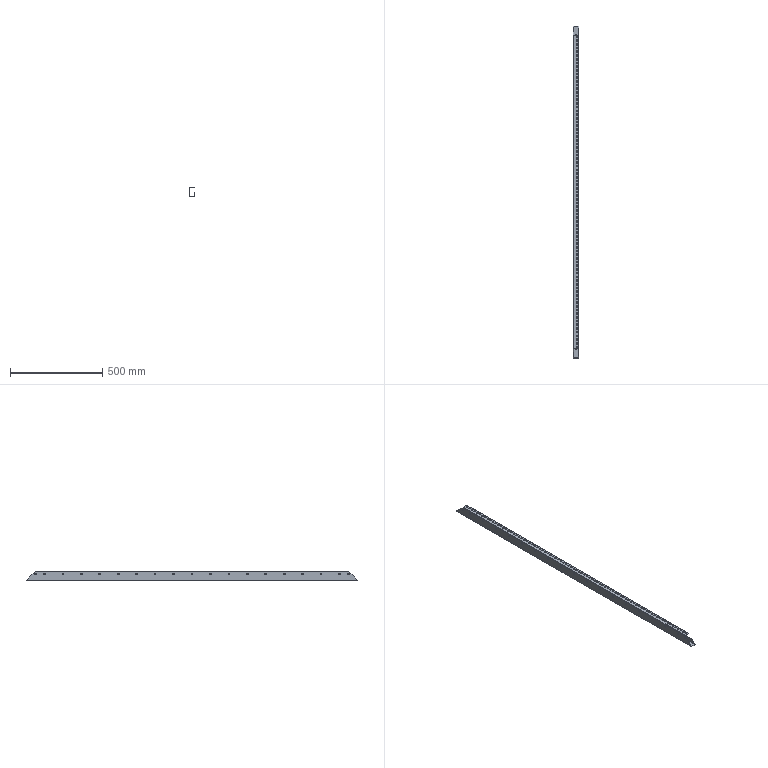Component | SolidWorks | KSHE-016.1.SLDPRT-1_KSHE-016.002-1 | 1 solid | 256 faces | volume 434150 mm3 | cylinder 222 | plane 30 | spline 4 | commonest cylinder face diameters 9 x208 5.1 x8 4.2 x3 0.2 x3